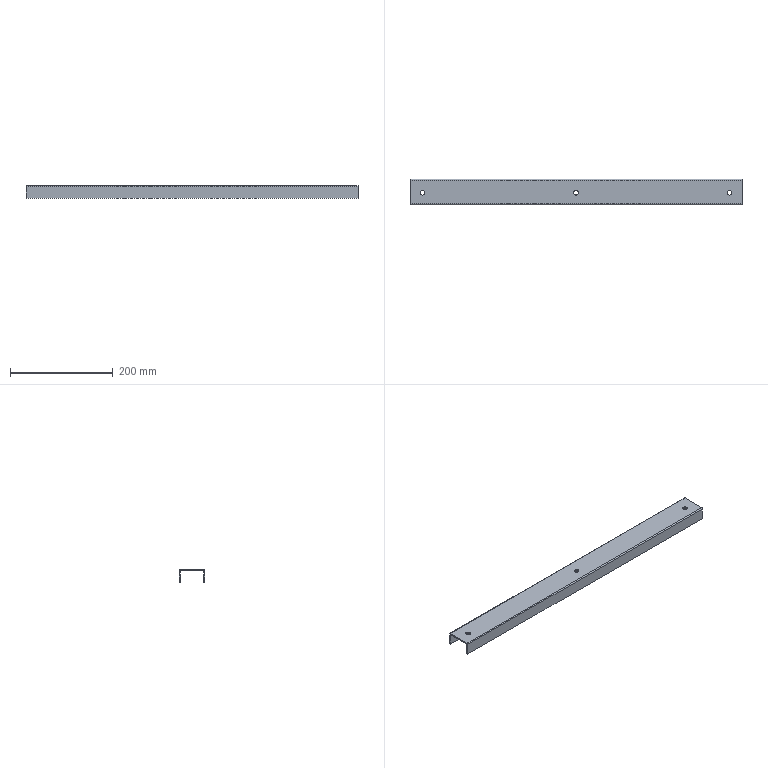Component | SolidWorks | FrameAssembly-1_FrameWeldment-1_MiddleBendPlate-1 | 1 solid | 18 faces | box 645 x 50 x 25 mm | volume 151603 mm3 | plane 10 | cylinder 8 | commonest cylinder face diameters 9 x6 4 x2
STEP:
#1=COLOUR_RGB('',0.7922,0.8196,0.9333);
#2=FILL_AREA_STYLE_COLOUR('',#1);
#3=FILL_AREA_STYLE('',(#2));
#4=SURFACE_STYLE_FILL_AREA(#3);
#5=SURFACE_SIDE_STYLE('',(#4));
#6=SURFACE_STYLE_USAGE(.BOTH.,#5);
#7=PRESENTATION_STYLE_ASSIGNMENT((#6));
#8=CARTESIAN_POINT('',(-11.585,-2.84,-1.339));
#9=VERTEX_POINT('',#8);
#10=CARTESIAN_POINT('',(-11.939,-2.84,-1.339));
#11=VERTEX_POINT('',#10);
#12=CARTESIAN_POINT('',(-11.762,-2.84,-1.339));
#13=DIRECTION('',(0.,-0.,1.));
#14=DIRECTION('',(-1.,0.,0.));
#15=AXIS2_PLACEMENT_3D('',#12,#13,#14);
#16=CIRCLE('',#15,0.1772);
#17=EDGE_CURVE('',#9,#11,#16,.T.);
#18=ORIENTED_EDGE('',*,*,#17,.F.);
#19=CARTESIAN_POINT('',(-11.585,-2.84,-1.24));
#20=VERTEX_POINT('',#19);
#21=CARTESIAN_POINT('',(-11.585,-2.84,-1.24));
#22=DIRECTION('',(0.,-0.,1.));
#23=VECTOR('',#22,39.37);
#24=LINE('',#21,#23);
#25=EDGE_CURVE('',#9,#20,#24,.T.);
#26=ORIENTED_EDGE('',*,*,#25,.T.);
#27=CARTESIAN_POINT('',(-11.939,-2.84,-1.24));
#28=VERTEX_POINT('',#27);
#29=CARTESIAN_POINT('',(-11.762,-2.84,-1.24));
#30=DIRECTION('',(0.,-0.,1.));
#31=DIRECTION('',(-1.,0.,0.));
#32=AXIS2_PLACEMENT_3D('',#29,#30,#31);
#33=CIRCLE('',#32,0.1772);
#34=EDGE_CURVE('',#20,#28,#33,.T.);
#35=ORIENTED_EDGE('',*,*,#34,.T.);
#36=CARTESIAN_POINT('',(-11.939,-2.84,-1.24));
#37=DIRECTION('',(0.,-0.,1.));
#38=VECTOR('',#37,39.37);
#39=LINE('',#36,#38);
#40=EDGE_CURVE('',#11,#28,#39,.T.);
#41=ORIENTED_EDGE('',*,*,#40,.F.);
#42=EDGE_LOOP('',(#18,#26,#35,#41));
#43=FACE_OUTER_BOUND('',#42,.T.);
#44=CARTESIAN_POINT('',(-11.762,-2.84,-1.24));
#45=DIRECTION('',(0.,-0.,1.));
#46=DIRECTION('',(-1.,0.,0.));
#47=AXIS2_PLACEMENT_3D('',#44,#45,#46);
#48=CYLINDRICAL_SURFACE('',#47,0.1772);
#49=ADVANCED_FACE('',(#43),#48,.F.);
#50=CARTESIAN_POINT('',(-23.317,-2.84,-1.339));
#51=VERTEX_POINT('',#50);
#52=CARTESIAN_POINT('',(-23.671,-2.84,-1.339));
#53=VERTEX_POINT('',#52);
#54=CARTESIAN_POINT('',(-23.494,-2.84,-1.339));
#55=DIRECTION('',(0.,-0.,1.));
#56=DIRECTION('',(-1.,0.,0.));
#57=AXIS2_PLACEMENT_3D('',#54,#55,#56);
#58=CIRCLE('',#57,0.1772);
#59=EDGE_CURVE('',#51,#53,#58,.T.);
#60=ORIENTED_EDGE('',*,*,#59,.F.);
#61=CARTESIAN_POINT('',(-23.317,-2.84,-1.24));
#62=VERTEX_POINT('',#61);
#63=CARTESIAN_POINT('',(-23.317,-2.84,-1.24));
#64=DIRECTION('',(0.,-0.,1.));
#65=VECTOR('',#64,39.37);
#66=LINE('',#63,#65);
#67=EDGE_CURVE('',#51,#62,#66,.T.);
#68=ORIENTED_EDGE('',*,*,#67,.T.);
#69=CARTESIAN_POINT('',(-23.671,-2.84,-1.24));
#70=VERTEX_POINT('',#69);
#71=CARTESIAN_POINT('',(-23.494,-2.84,-1.24));
#72=DIRECTION('',(0.,-0.,1.));
#73=DIRECTION('',(-1.,0.,0.));
#74=AXIS2_PLACEMENT_3D('',#71,#72,#73);
#75=CIRCLE('',#74,0.1772);
#76=EDGE_CURVE('',#62,#70,#75,.T.);
#77=ORIENTED_EDGE('',*,*,#76,.T.);
#78=CARTESIAN_POINT('',(-23.671,-2.84,-1.24));
#79=DIRECTION('',(0.,-0.,1.));
#80=VECTOR('',#79,39.37);
#81=LINE('',#78,#80);
#82=EDGE_CURVE('',#53,#70,#81,.T.);
#83=ORIENTED_EDGE('',*,*,#82,.F.);
#84=EDGE_LOOP('',(#60,#68,#77,#83));
#85=FACE_OUTER_BOUND('',#84,.T.);
#86=CARTESIAN_POINT('',(-23.494,-2.84,-1.24));
#87=DIRECTION('',(0.,-0.,1.));
#88=DIRECTION('',(-1.,0.,0.));
#89=AXIS2_PLACEMENT_3D('',#86,#87,#88);
#90=CYLINDRICAL_SURFACE('',#89,0.1772);
#91=ADVANCED_FACE('',(#85),#90,.F.);
#92=CARTESIAN_POINT('',(0.1478,-2.84,-1.339));
#93=VERTEX_POINT('',#92);
#94=CARTESIAN_POINT('',(-0.2065,-2.84,-1.339));
#95=VERTEX_POINT('',#94);
#96=CARTESIAN_POINT('',(-0.02938,-2.84,-1.339));
#97=DIRECTION('',(0.,-0.,1.));
#98=DIRECTION('',(-1.,0.,0.));
#99=AXIS2_PLACEMENT_3D('',#96,#97,#98);
#100=CIRCLE('',#99,0.1772);
#101=EDGE_CURVE('',#93,#95,#100,.T.);
#102=ORIENTED_EDGE('',*,*,#101,.F.);
#103=CARTESIAN_POINT('',(0.1478,-2.84,-1.24));
#104=VERTEX_POINT('',#103);
#105=CARTESIAN_POINT('',(0.1478,-2.84,-1.24));
#106=DIRECTION('',(0.,-0.,1.));
#107=VECTOR('',#106,39.37);
#108=LINE('',#105,#107);
#109=EDGE_CURVE('',#93,#104,#108,.T.);
#110=ORIENTED_EDGE('',*,*,#109,.T.);
#111=CARTESIAN_POINT('',(-0.2065,-2.84,-1.24));
#112=VERTEX_POINT('',#111);
#113=CARTESIAN_POINT('',(-0.02938,-2.84,-1.24));
#114=DIRECTION('',(0.,-0.,1.));
#115=DIRECTION('',(-1.,0.,0.));
#116=AXIS2_PLACEMENT_3D('',#113,#114,#115);
#117=CIRCLE('',#116,0.1772);
#118=EDGE_CURVE('',#104,#112,#117,.T.);
#119=ORIENTED_EDGE('',*,*,#118,.T.);
#120=CARTESIAN_POINT('',(-0.2065,-2.84,-1.24));
#121=DIRECTION('',(0.,-0.,1.));
#122=VECTOR('',#121,39.37);
#123=LINE('',#120,#122);
#124=EDGE_CURVE('',#95,#112,#123,.T.);
#125=ORIENTED_EDGE('',*,*,#124,.F.);
#126=EDGE_LOOP('',(#102,#110,#119,#125));
#127=FACE_OUTER_BOUND('',#126,.T.);
#128=CARTESIAN_POINT('',(-0.02938,-2.84,-1.24));
#129=DIRECTION('',(0.,-0.,1.));
#130=DIRECTION('',(-1.,0.,0.));
#131=AXIS2_PLACEMENT_3D('',#128,#129,#130);
#132=CYLINDRICAL_SURFACE('',#131,0.1772);
#133=ADVANCED_FACE('',(#127),#132,.F.);
#134=CARTESIAN_POINT('',(0.9352,-1.895,-2.224));
#135=VERTEX_POINT('',#134);
#136=CARTESIAN_POINT('',(-24.459,-1.895,-2.224));
#137=VERTEX_POINT('',#136);
#138=CARTESIAN_POINT('',(0.9352,-1.895,-2.224));
#139=DIRECTION('',(-1.,0.,0.));
#140=VECTOR('',#139,39.37);
#141=LINE('',#138,#140);
#142=EDGE_CURVE('',#135,#137,#141,.T.);
#143=ORIENTED_EDGE('',*,*,#142,.T.);
#144=CARTESIAN_POINT('',(-24.459,-1.796,-2.224));
#145=VERTEX_POINT('',#144);
#146=CARTESIAN_POINT('',(-24.459,-3.765,-2.224));
#147=DIRECTION('',(0.,1.,0.));
#148=VECTOR('',#147,39.37);
#149=LINE('',#146,#148);
#150=EDGE_CURVE('',#137,#145,#149,.T.);
#151=ORIENTED_EDGE('',*,*,#150,.T.);
#152=CARTESIAN_POINT('',(0.9352,-1.796,-2.224));
#153=VERTEX_POINT('',#152);
#154=CARTESIAN_POINT('',(-24.459,-1.796,-2.224));
#155=DIRECTION('',(1.,-0.,-0.));
#156=VECTOR('',#155,39.37);
#157=LINE('',#154,#156);
#158=EDGE_CURVE('',#145,#153,#157,.T.);
#159=ORIENTED_EDGE('',*,*,#158,.T.);
#160=CARTESIAN_POINT('',(0.9352,-3.765,-2.224));
#161=DIRECTION('',(0.,1.,0.));
#162=VECTOR('',#161,39.37);
#163=LINE('',#160,#162);
#164=EDGE_CURVE('',#135,#153,#163,.T.);
#165=ORIENTED_EDGE('',*,*,#164,.F.);
#166=EDGE_LOOP('',(#143,#151,#159,#165));
#167=FACE_OUTER_BOUND('',#166,.T.);
#168=CARTESIAN_POINT('',(-24.459,-3.765,-2.224));
#169=DIRECTION('',(-0.,0.,-1.));
#170=DIRECTION('',(1.,-0.,-0.));
#171=AXIS2_PLACEMENT_3D('',#168,#169,#170);
#172=PLANE('',#171);
#173=ADVANCED_FACE('',(#167),#172,.T.);
#174=CARTESIAN_POINT('',(0.9352,-3.765,-1.319));
#175=VERTEX_POINT('',#174);
#176=CARTESIAN_POINT('',(0.9352,-3.765,-2.224));
#177=VERTEX_POINT('',#176);
#178=CARTESIAN_POINT('',(0.9352,-3.765,-1.319));
#179=DIRECTION('',(-0.,0.,-1.));
#180=VECTOR('',#179,39.37);
#181=LINE('',#178,#180);
#182=EDGE_CURVE('',#175,#177,#181,.T.);
#183=ORIENTED_EDGE('',*,*,#182,.F.);
#184=CARTESIAN_POINT('',(-24.459,-3.765,-1.319));
#185=VERTEX_POINT('',#184);
#186=CARTESIAN_POINT('',(-24.459,-3.765,-1.319));
#187=DIRECTION('',(1.,-0.,-0.));
#188=VECTOR('',#187,39.37);
#189=LINE('',#186,#188);
#190=EDGE_CURVE('',#185,#175,#189,.T.);
#191=ORIENTED_EDGE('',*,*,#190,.F.);
#192=CARTESIAN_POINT('',(-24.459,-3.765,-2.224));
#193=VERTEX_POINT('',#192);
#194=CARTESIAN_POINT('',(-24.459,-3.765,-1.319));
#195=DIRECTION('',(-0.,0.,-1.));
#196=VECTOR('',#195,39.37);
#197=LINE('',#194,#196);
#198=EDGE_CURVE('',#185,#193,#197,.T.);
#199=ORIENTED_EDGE('',*,*,#198,.T.);
#200=CARTESIAN_POINT('',(-24.459,-3.765,-2.224));
#201=DIRECTION('',(1.,-0.,-0.));
#202=VECTOR('',#201,39.37);
#203=LINE('',#200,#202);
#204=EDGE_CURVE('',#193,#177,#203,.T.);
#205=ORIENTED_EDGE('',*,*,#204,.T.);
#206=EDGE_LOOP('',(#183,#191,#199,#205));
#207=FACE_OUTER_BOUND('',#206,.T.);
#208=CARTESIAN_POINT('',(-24.459,-3.765,-1.319));
#209=DIRECTION('',(-0.,-1.,-0.));
#210=DIRECTION('',(-1.,0.,0.));
#211=AXIS2_PLACEMENT_3D('',#208,#209,#210);
#212=PLANE('',#211);
#213=ADVANCED_FACE('',(#207),#212,.T.);
#214=CARTESIAN_POINT('',(0.9352,-3.686,-1.24));
#215=VERTEX_POINT('',#214);
#216=CARTESIAN_POINT('',(0.9352,-3.686,-1.319));
#217=DIRECTION('',(1.,-0.,-0.));
#218=DIRECTION('',(0.,0.,1.));
#219=AXIS2_PLACEMENT_3D('',#216,#217,#218);
#220=CIRCLE('',#219,0.07874);
#221=EDGE_CURVE('',#215,#175,#220,.T.);
#222=ORIENTED_EDGE('',*,*,#221,.F.);
#223=CARTESIAN_POINT('',(-24.459,-3.686,-1.24));
#224=VERTEX_POINT('',#223);
#225=CARTESIAN_POINT('',(-24.459,-3.686,-1.24));
#226=DIRECTION('',(1.,-0.,-0.));
#227=VECTOR('',#226,39.37);
#228=LINE('',#225,#227);
#229=EDGE_CURVE('',#224,#215,#228,.T.);
#230=ORIENTED_EDGE('',*,*,#229,.F.);
#231=CARTESIAN_POINT('',(-24.459,-3.686,-1.319));
#232=DIRECTION('',(1.,-0.,-0.));
#233=DIRECTION('',(0.,0.,1.));
#234=AXIS2_PLACEMENT_3D('',#231,#232,#233);
#235=CIRCLE('',#234,0.07874);
#236=EDGE_CURVE('',#224,#185,#235,.T.);
#237=ORIENTED_EDGE('',*,*,#236,.T.);
#238=ORIENTED_EDGE('',*,*,#190,.T.);
#239=EDGE_LOOP('',(#222,#230,#237,#238));
#240=FACE_OUTER_BOUND('',#239,.T.);
#241=CARTESIAN_POINT('',(-24.459,-3.686,-1.319));
#242=DIRECTION('',(1.,-0.,-0.));
#243=DIRECTION('',(0.,0.,1.));
#244=AXIS2_PLACEMENT_3D('',#241,#242,#243);
#245=CYLINDRICAL_SURFACE('',#244,0.07874);
#246=ADVANCED_FACE('',(#240),#245,.T.);
#247=CARTESIAN_POINT('',(-11.762,-2.84,-1.24));
#248=DIRECTION('',(0.,-0.,1.));
#249=DIRECTION('',(-1.,0.,0.));
#250=AXIS2_PLACEMENT_3D('',#247,#248,#249);
#251=CIRCLE('',#250,0.1772);
#252=EDGE_CURVE('',#28,#20,#251,.T.);
#253=ORIENTED_EDGE('',*,*,#252,.F.);
#254=ORIENTED_EDGE('',*,*,#34,.F.);
#255=EDGE_LOOP('',(#253,#254));
#256=FACE_BOUND('',#255,.T.);
#257=CARTESIAN_POINT('',(-23.494,-2.84,-1.24));
#258=DIRECTION('',(0.,-0.,1.));
#259=DIRECTION('',(-1.,0.,0.));
#260=AXIS2_PLACEMENT_3D('',#257,#258,#259);
#261=CIRCLE('',#260,0.1772);
#262=EDGE_CURVE('',#70,#62,#261,.T.);
#263=ORIENTED_EDGE('',*,*,#262,.F.);
#264=ORIENTED_EDGE('',*,*,#76,.F.);
#265=EDGE_LOOP('',(#263,#264));
#266=FACE_BOUND('',#265,.T.);
#267=CARTESIAN_POINT('',(-0.02938,-2.84,-1.24));
#268=DIRECTION('',(0.,-0.,1.));
#269=DIRECTION('',(-1.,0.,0.));
#270=AXIS2_PLACEMENT_3D('',#267,#268,#269);
#271=CIRCLE('',#270,0.1772);
#272=EDGE_CURVE('',#112,#104,#271,.T.);
#273=ORIENTED_EDGE('',*,*,#272,.F.);
#274=ORIENTED_EDGE('',*,*,#118,.F.);
#275=EDGE_LOOP('',(#273,#274));
#276=FACE_BOUND('',#275,.T.);
#277=CARTESIAN_POINT('',(0.9352,-1.875,-1.24));
#278=VERTEX_POINT('',#277);
#279=CARTESIAN_POINT('',(0.9352,-1.875,-1.24));
#280=DIRECTION('',(-0.,-1.,0.));
#281=VECTOR('',#280,39.37);
#282=LINE('',#279,#281);
#283=EDGE_CURVE('',#278,#215,#282,.T.);
#284=ORIENTED_EDGE('',*,*,#283,.F.);
#285=CARTESIAN_POINT('',(-24.459,-1.875,-1.24));
#286=VERTEX_POINT('',#285);
#287=CARTESIAN_POINT('',(-24.459,-1.875,-1.24));
#288=DIRECTION('',(1.,-0.,-0.));
#289=VECTOR('',#288,39.37);
#290=LINE('',#287,#289);
#291=EDGE_CURVE('',#286,#278,#290,.T.);
#292=ORIENTED_EDGE('',*,*,#291,.F.);
#293=CARTESIAN_POINT('',(-24.459,-1.875,-1.24));
#294=DIRECTION('',(-0.,-1.,0.));
#295=VECTOR('',#294,39.37);
#296=LINE('',#293,#295);
#297=EDGE_CURVE('',#286,#224,#296,.T.);
#298=ORIENTED_EDGE('',*,*,#297,.T.);
#299=ORIENTED_EDGE('',*,*,#229,.T.);
#300=EDGE_LOOP('',(#284,#292,#298,#299));
#301=FACE_OUTER_BOUND('',#300,.T.);
#302=CARTESIAN_POINT('',(-24.459,-1.875,-1.24));
#303=DIRECTION('',(0.,0.,1.));
#304=DIRECTION('',(0.,1.,-0.));
#305=AXIS2_PLACEMENT_3D('',#302,#303,#304);
#306=PLANE('',#305);
#307=ADVANCED_FACE('',(#256,#266,#276,#301),#306,.T.);
#308=CARTESIAN_POINT('',(0.9352,-1.796,-1.319));
#309=VERTEX_POINT('',#308);
#310=CARTESIAN_POINT('',(0.9352,-1.875,-1.319));
#311=DIRECTION('',(1.,-0.,-0.));
#312=DIRECTION('',(0.,0.,1.));
#313=AXIS2_PLACEMENT_3D('',#310,#311,#312);
#314=CIRCLE('',#313,0.07874);
#315=EDGE_CURVE('',#309,#278,#314,.T.);
#316=ORIENTED_EDGE('',*,*,#315,.F.);
#317=CARTESIAN_POINT('',(-24.459,-1.796,-1.319));
#318=VERTEX_POINT('',#317);
#319=CARTESIAN_POINT('',(-24.459,-1.796,-1.319));
#320=DIRECTION('',(1.,-0.,-0.));
#321=VECTOR('',#320,39.37);
#322=LINE('',#319,#321);
#323=EDGE_CURVE('',#318,#309,#322,.T.);
#324=ORIENTED_EDGE('',*,*,#323,.F.);
#325=CARTESIAN_POINT('',(-24.459,-1.875,-1.319));
#326=DIRECTION('',(1.,-0.,-0.));
#327=DIRECTION('',(0.,0.,1.));
#328=AXIS2_PLACEMENT_3D('',#325,#326,#327);
#329=CIRCLE('',#328,0.07874);
#330=EDGE_CURVE('',#318,#286,#329,.T.);
#331=ORIENTED_EDGE('',*,*,#330,.T.);
#332=ORIENTED_EDGE('',*,*,#291,.T.);
#333=EDGE_LOOP('',(#316,#324,#331,#332));
#334=FACE_OUTER_BOUND('',#333,.T.);
#335=CARTESIAN_POINT('',(-24.459,-1.875,-1.319));
#336=DIRECTION('',(1.,-0.,-0.));
#337=DIRECTION('',(0.,0.,1.));
#338=AXIS2_PLACEMENT_3D('',#335,#336,#337);
#339=CYLINDRICAL_SURFACE('',#338,0.07874);
#340=ADVANCED_FACE('',(#334),#339,.T.);
#341=CARTESIAN_POINT('',(0.9352,-1.796,-2.224));
#342=DIRECTION('',(0.,-0.,1.));
#343=VECTOR('',#342,39.37);
#344=LINE('',#341,#343);
#345=EDGE_CURVE('',#153,#309,#344,.T.);
#346=ORIENTED_EDGE('',*,*,#345,.F.);
#347=ORIENTED_EDGE('',*,*,#158,.F.);
#348=CARTESIAN_POINT('',(-24.459,-1.796,-2.224));
#349=DIRECTION('',(0.,-0.,1.));
#350=VECTOR('',#349,39.37);
#351=LINE('',#348,#350);
#352=EDGE_CURVE('',#145,#318,#351,.T.);
#353=ORIENTED_EDGE('',*,*,#352,.T.);
#354=ORIENTED_EDGE('',*,*,#323,.T.);
#355=EDGE_LOOP('',(#346,#347,#353,#354));
#356=FACE_OUTER_BOUND('',#355,.T.);
#357=CARTESIAN_POINT('',(-24.459,-1.796,-2.224));
#358=DIRECTION('',(0.,1.,0.));
#359=DIRECTION('',(1.,-0.,-0.));
#360=AXIS2_PLACEMENT_3D('',#357,#358,#359);
#361=PLANE('',#360);
#362=ADVANCED_FACE('',(#356),#361,.T.);
#363=CARTESIAN_POINT('',(0.9352,-3.666,-2.224));
#364=VERTEX_POINT('',#363);
#365=CARTESIAN_POINT('',(-24.459,-3.666,-2.224));
#366=VERTEX_POINT('',#365);
#367=CARTESIAN_POINT('',(0.9352,-3.666,-2.224));
#368=DIRECTION('',(-1.,0.,0.));
#369=VECTOR('',#368,39.37);
#370=LINE('',#367,#369);
#371=EDGE_CURVE('',#364,#366,#370,.T.);
#372=ORIENTED_EDGE('',*,*,#371,.F.);
#373=CARTESIAN_POINT('',(0.9352,-3.765,-2.224));
#374=DIRECTION('',(0.,1.,0.));
#375=VECTOR('',#374,39.37);
#376=LINE('',#373,#375);
#377=EDGE_CURVE('',#177,#364,#376,.T.);
#378=ORIENTED_EDGE('',*,*,#377,.F.);
#379=ORIENTED_EDGE('',*,*,#204,.F.);
#380=CARTESIAN_POINT('',(-24.459,-3.765,-2.224));
#381=DIRECTION('',(0.,1.,0.));
#382=VECTOR('',#381,39.37);
#383=LINE('',#380,#382);
#384=EDGE_CURVE('',#193,#366,#383,.T.);
#385=ORIENTED_EDGE('',*,*,#384,.T.);
#386=EDGE_LOOP('',(#372,#378,#379,#385));
#387=FACE_OUTER_BOUND('',#386,.T.);
#388=CARTESIAN_POINT('',(-24.459,-3.765,-2.224));
#389=DIRECTION('',(-0.,0.,-1.));
#390=DIRECTION('',(1.,-0.,-0.));
#391=AXIS2_PLACEMENT_3D('',#388,#389,#390);
#392=PLANE('',#391);
#393=ADVANCED_FACE('',(#387),#392,.T.);
#394=ORIENTED_EDGE('',*,*,#150,.F.);
#395=CARTESIAN_POINT('',(-24.459,-1.895,-1.339));
#396=VERTEX_POINT('',#395);
#397=CARTESIAN_POINT('',(-24.459,-1.895,-1.339));
#398=DIRECTION('',(-0.,0.,-1.));
#399=VECTOR('',#398,39.37);
#400=LINE('',#397,#399);
#401=EDGE_CURVE('',#396,#137,#400,.T.);
#402=ORIENTED_EDGE('',*,*,#401,.F.);
#403=CARTESIAN_POINT('',(-24.459,-3.666,-1.339));
#404=VERTEX_POINT('',#403);
#405=CARTESIAN_POINT('',(-24.459,-3.666,-1.339));
#406=DIRECTION('',(0.,1.,0.));
#407=VECTOR('',#406,39.37);
#408=LINE('',#405,#407);
#409=EDGE_CURVE('',#404,#396,#408,.T.);
#410=ORIENTED_EDGE('',*,*,#409,.F.);
#411=CARTESIAN_POINT('',(-24.459,-3.666,-2.224));
#412=DIRECTION('',(0.,-0.,1.));
#413=VECTOR('',#412,39.37);
#414=LINE('',#411,#413);
#415=EDGE_CURVE('',#366,#404,#414,.T.);
#416=ORIENTED_EDGE('',*,*,#415,.F.);
#417=ORIENTED_EDGE('',*,*,#384,.F.);
#418=ORIENTED_EDGE('',*,*,#198,.F.);
#419=ORIENTED_EDGE('',*,*,#236,.F.);
#420=ORIENTED_EDGE('',*,*,#297,.F.);
#421=ORIENTED_EDGE('',*,*,#330,.F.);
#422=ORIENTED_EDGE('',*,*,#352,.F.);
#423=EDGE_LOOP('',(#394,#402,#410,#416,#417,#418,#419,#420,#421,#422));
#424=FACE_OUTER_BOUND('',#423,.T.);
#425=CARTESIAN_POINT('',(-24.459,-1.875,-1.319));
#426=DIRECTION('',(1.,-0.,-0.));
#427=DIRECTION('',(0.,-0.,1.));
#428=AXIS2_PLACEMENT_3D('',#425,#426,#427);
#429=PLANE('',#428);
#430=ADVANCED_FACE('',(#424),#429,.F.);
#431=CARTESIAN_POINT('',(0.9352,-1.895,-1.339));
#432=VERTEX_POINT('',#431);
#433=CARTESIAN_POINT('',(0.9352,-1.895,-1.339));
#434=DIRECTION('',(-0.,0.,-1.));
#435=VECTOR('',#434,39.37);
#436=LINE('',#433,#435);
#437=EDGE_CURVE('',#432,#135,#436,.T.);
#438=ORIENTED_EDGE('',*,*,#437,.T.);
#439=ORIENTED_EDGE('',*,*,#164,.T.);
#440=ORIENTED_EDGE('',*,*,#345,.T.);
#441=ORIENTED_EDGE('',*,*,#315,.T.);
#442=ORIENTED_EDGE('',*,*,#283,.T.);
#443=ORIENTED_EDGE('',*,*,#221,.T.);
#444=ORIENTED_EDGE('',*,*,#182,.T.);
#445=ORIENTED_EDGE('',*,*,#377,.T.);
#446=CARTESIAN_POINT('',(0.9352,-3.666,-1.339));
#447=VERTEX_POINT('',#446);
#448=CARTESIAN_POINT('',(0.9352,-3.666,-2.224));
#449=DIRECTION('',(0.,-0.,1.));
#450=VECTOR('',#449,39.37);
#451=LINE('',#448,#450);
#452=EDGE_CURVE('',#364,#447,#451,.T.);
#453=ORIENTED_EDGE('',*,*,#452,.T.);
#454=CARTESIAN_POINT('',(0.9352,-3.666,-1.339));
#455=DIRECTION('',(0.,1.,0.));
#456=VECTOR('',#455,39.37);
#457=LINE('',#454,#456);
#458=EDGE_CURVE('',#447,#432,#457,.T.);
#459=ORIENTED_EDGE('',*,*,#458,.T.);
#460=EDGE_LOOP('',(#438,#439,#440,#441,#442,#443,#444,#445,#453,#459));
#461=FACE_OUTER_BOUND('',#460,.T.);
#462=CARTESIAN_POINT('',(0.9352,-1.875,-1.319));
#463=DIRECTION('',(1.,-0.,-0.));
#464=DIRECTION('',(0.,-0.,1.));
#465=AXIS2_PLACEMENT_3D('',#462,#463,#464);
#466=PLANE('',#465);
#467=ADVANCED_FACE('',(#461),#466,.T.);
#468=ORIENTED_EDGE('',*,*,#401,.T.);
#469=ORIENTED_EDGE('',*,*,#142,.F.);
#470=ORIENTED_EDGE('',*,*,#437,.F.);
#471=CARTESIAN_POINT('',(0.9352,-1.895,-1.339));
#472=DIRECTION('',(-1.,0.,0.));
#473=VECTOR('',#472,39.37);
#474=LINE('',#471,#473);
#475=EDGE_CURVE('',#432,#396,#474,.T.);
#476=ORIENTED_EDGE('',*,*,#475,.T.);
#477=EDGE_LOOP('',(#468,#469,#470,#476));
#478=FACE_OUTER_BOUND('',#477,.T.);
#479=CARTESIAN_POINT('',(0.9352,-1.895,-1.339));
#480=DIRECTION('',(0.,1.,0.));
#481=DIRECTION('',(1.,-0.,-0.));
#482=AXIS2_PLACEMENT_3D('',#479,#480,#481);
#483=PLANE('',#482);
#484=ADVANCED_FACE('',(#478),#483,.F.);
#485=CARTESIAN_POINT('',(-11.762,-2.84,-1.339));
#486=DIRECTION('',(0.,-0.,1.));
#487=DIRECTION('',(-1.,0.,0.));
#488=AXIS2_PLACEMENT_3D('',#485,#486,#487);
#489=CIRCLE('',#488,0.1772);
#490=EDGE_CURVE('',#11,#9,#489,.T.);
#491=ORIENTED_EDGE('',*,*,#490,.T.);
#492=ORIENTED_EDGE('',*,*,#17,.T.);
#493=EDGE_LOOP('',(#491,#492));
#494=FACE_BOUND('',#493,.T.);
#495=CARTESIAN_POINT('',(-23.494,-2.84,-1.339));
#496=DIRECTION('',(0.,-0.,1.));
#497=DIRECTION('',(-1.,0.,0.));
#498=AXIS2_PLACEMENT_3D('',#495,#496,#497);
#499=CIRCLE('',#498,0.1772);
#500=EDGE_CURVE('',#53,#51,#499,.T.);
#501=ORIENTED_EDGE('',*,*,#500,.T.);
#502=ORIENTED_EDGE('',*,*,#59,.T.);
#503=EDGE_LOOP('',(#501,#502));
#504=FACE_BOUND('',#503,.T.);
#505=CARTESIAN_POINT('',(-0.02938,-2.84,-1.339));
#506=DIRECTION('',(0.,-0.,1.));
#507=DIRECTION('',(-1.,0.,0.));
#508=AXIS2_PLACEMENT_3D('',#505,#506,#507);
#509=CIRCLE('',#508,0.1772);
#510=EDGE_CURVE('',#95,#93,#509,.T.);
#511=ORIENTED_EDGE('',*,*,#510,.T.);
#512=ORIENTED_EDGE('',*,*,#101,.T.);
#513=EDGE_LOOP('',(#511,#512));
#514=FACE_BOUND('',#513,.T.);
#515=ORIENTED_EDGE('',*,*,#409,.T.);
#516=ORIENTED_EDGE('',*,*,#475,.F.);
#517=ORIENTED_EDGE('',*,*,#458,.F.);
#518=CARTESIAN_POINT('',(0.9352,-3.666,-1.339));
#519=DIRECTION('',(-1.,0.,0.));
#520=VECTOR('',#519,39.37);
#521=LINE('',#518,#520);
#522=EDGE_CURVE('',#447,#404,#521,.T.);
#523=ORIENTED_EDGE('',*,*,#522,.T.);
#524=EDGE_LOOP('',(#515,#516,#517,#523));
#525=FACE_OUTER_BOUND('',#524,.T.);
#526=CARTESIAN_POINT('',(0.9352,-3.666,-1.339));
#527=DIRECTION('',(0.,-0.,1.));
#528=DIRECTION('',(-1.,0.,0.));
#529=AXIS2_PLACEMENT_3D('',#526,#527,#528);
#530=PLANE('',#529);
#531=ADVANCED_FACE('',(#494,#504,#514,#525),#530,.F.);
#532=ORIENTED_EDGE('',*,*,#415,.T.);
#533=ORIENTED_EDGE('',*,*,#522,.F.);
#534=ORIENTED_EDGE('',*,*,#452,.F.);
#535=ORIENTED_EDGE('',*,*,#371,.T.);
#536=EDGE_LOOP('',(#532,#533,#534,#535));
#537=FACE_OUTER_BOUND('',#536,.T.);
#538=CARTESIAN_POINT('',(0.9352,-3.666,-2.224));
#539=DIRECTION('',(-0.,-1.,-0.));
#540=DIRECTION('',(-1.,0.,0.));
#541=AXIS2_PLACEMENT_3D('',#538,#539,#540);
#542=PLANE('',#541);
#543=ADVANCED_FACE('',(#537),#542,.F.);
#544=ORIENTED_EDGE('',*,*,#109,.F.);
#545=ORIENTED_EDGE('',*,*,#510,.F.);
#546=ORIENTED_EDGE('',*,*,#124,.T.);
#547=ORIENTED_EDGE('',*,*,#272,.T.);
#548=EDGE_LOOP('',(#544,#545,#546,#547));
#549=FACE_OUTER_BOUND('',#548,.T.);
#550=CARTESIAN_POINT('',(-0.02938,-2.84,-1.24));
#551=DIRECTION('',(0.,-0.,1.));
#552=DIRECTION('',(-1.,0.,0.));
#553=AXIS2_PLACEMENT_3D('',#550,#551,#552);
#554=CYLINDRICAL_SURFACE('',#553,0.1772);
#555=ADVANCED_FACE('',(#549),#554,.F.);
#556=ORIENTED_EDGE('',*,*,#67,.F.);
#557=ORIENTED_EDGE('',*,*,#500,.F.);
#558=ORIENTED_EDGE('',*,*,#82,.T.);
#559=ORIENTED_EDGE('',*,*,#262,.T.);
#560=EDGE_LOOP('',(#556,#557,#558,#559));
#561=FACE_OUTER_BOUND('',#560,.T.);
#562=CARTESIAN_POINT('',(-23.494,-2.84,-1.24));
#563=DIRECTION('',(0.,-0.,1.));
#564=DIRECTION('',(-1.,0.,0.));
#565=AXIS2_PLACEMENT_3D('',#562,#563,#564);
#566=CYLINDRICAL_SURFACE('',#565,0.1772);
#567=ADVANCED_FACE('',(#561),#566,.F.);
#568=ORIENTED_EDGE('',*,*,#25,.F.);
#569=ORIENTED_EDGE('',*,*,#490,.F.);
#570=ORIENTED_EDGE('',*,*,#40,.T.);
#571=ORIENTED_EDGE('',*,*,#252,.T.);
#572=EDGE_LOOP('',(#568,#569,#570,#571));
#573=FACE_OUTER_BOUND('',#572,.T.);
#574=CARTESIAN_POINT('',(-11.762,-2.84,-1.24));
#575=DIRECTION('',(0.,-0.,1.));
#576=DIRECTION('',(-1.,0.,0.));
#577=AXIS2_PLACEMENT_3D('',#574,#575,#576);
#578=CYLINDRICAL_SURFACE('',#577,0.1772);
#579=ADVANCED_FACE('',(#573),#578,.F.);
#580=CLOSED_SHELL('',(#49,#91,#133,#173,#213,#246,#307,#340,#362,#393,#430,#467,#484,#531,#543,#555,#567,#579));
#581=MANIFOLD_SOLID_BREP('',#580);
#582=STYLED_ITEM('',(#7),#581);
#583=PRESENTATION_LAYER_ASSIGNMENT('','',(#582));
#584=(LENGTH_UNIT()NAMED_UNIT(*)SI_UNIT($,.METRE.));
#585=LENGTH_MEASURE_WITH_UNIT(LENGTH_MEASURE(0.0254),#584);
#586=DIMENSIONAL_EXPONENTS(1.,0.,0.,0.,0.,0.,0.);
#587=(CONVERSION_BASED_UNIT('',#585)LENGTH_UNIT()NAMED_UNIT(#586));
#588=UNCERTAINTY_MEASURE_WITH_UNIT(LENGTH_MEASURE(0.00001),#587,'','');
#589=(NAMED_UNIT(*)PLANE_ANGLE_UNIT()SI_UNIT($,.RADIAN.));
#590=(NAMED_UNIT(*)SI_UNIT($,.STERADIAN.)SOLID_ANGLE_UNIT());
#591=(GEOMETRIC_REPRESENTATION_CONTEXT(3)GLOBAL_UNCERTAINTY_ASSIGNED_CONTEXT((#588))GLOBAL_UNIT_ASSIGNED_CONTEXT((#587,#589,#590))REPRESENTATION_CONTEXT('',''));
#592=MECHANICAL_DESIGN_GEOMETRIC_PRESENTATION_REPRESENTATION('',(#582),#591);
#593=CARTESIAN_POINT('',(0.,0.,0.));
#594=DIRECTION('',(0.,0.,1.));
#595=DIRECTION('',(1.,0.,0.));
#596=AXIS2_PLACEMENT_3D('',#593,#594,#595);
#597=(LENGTH_UNIT()NAMED_UNIT(*)SI_UNIT($,.METRE.));
#598=LENGTH_MEASURE_WITH_UNIT(LENGTH_MEASURE(0.0254),#597);
#599=DIMENSIONAL_EXPONENTS(1.,0.,0.,0.,0.,0.,0.);
#600=(CONVERSION_BASED_UNIT('',#598)LENGTH_UNIT()NAMED_UNIT(#599));
#601=UNCERTAINTY_MEASURE_WITH_UNIT(LENGTH_MEASURE(0.00001),#600,'','');
#602=(NAMED_UNIT(*)PLANE_ANGLE_UNIT()SI_UNIT($,.RADIAN.));
#603=(NAMED_UNIT(*)SI_UNIT($,.STERADIAN.)SOLID_ANGLE_UNIT());
#604=(GEOMETRIC_REPRESENTATION_CONTEXT(3)GLOBAL_UNCERTAINTY_ASSIGNED_CONTEXT((#601))GLOBAL_UNIT_ASSIGNED_CONTEXT((#600,#602,#603))REPRESENTATION_CONTEXT('',''));
#605=ADVANCED_BREP_SHAPE_REPRESENTATION('',(#581,#596),#604);